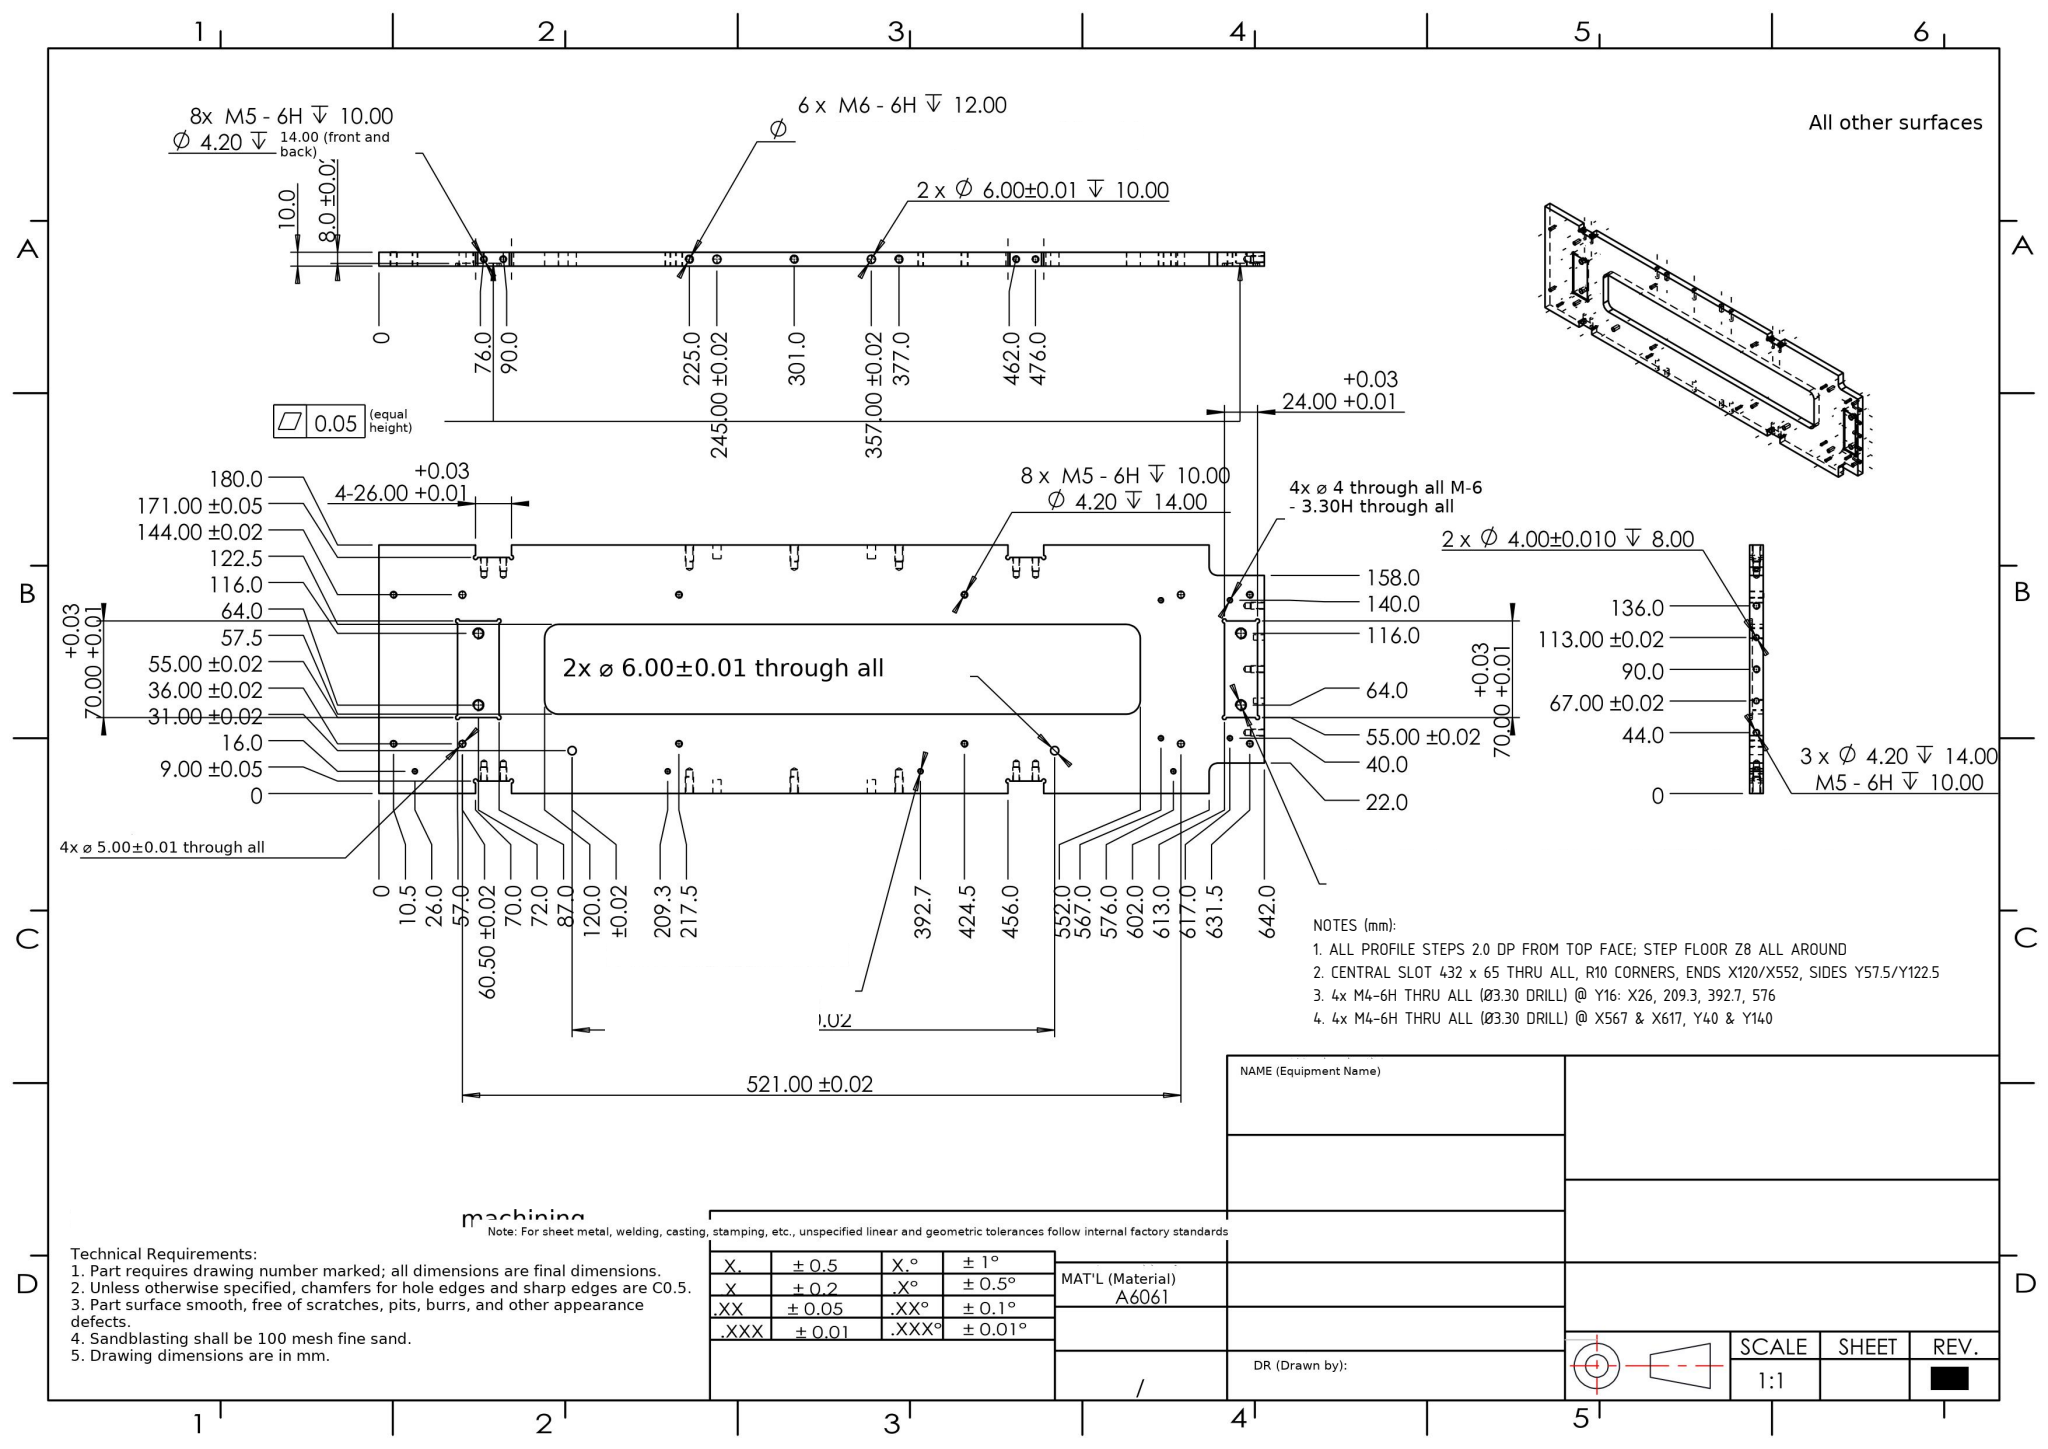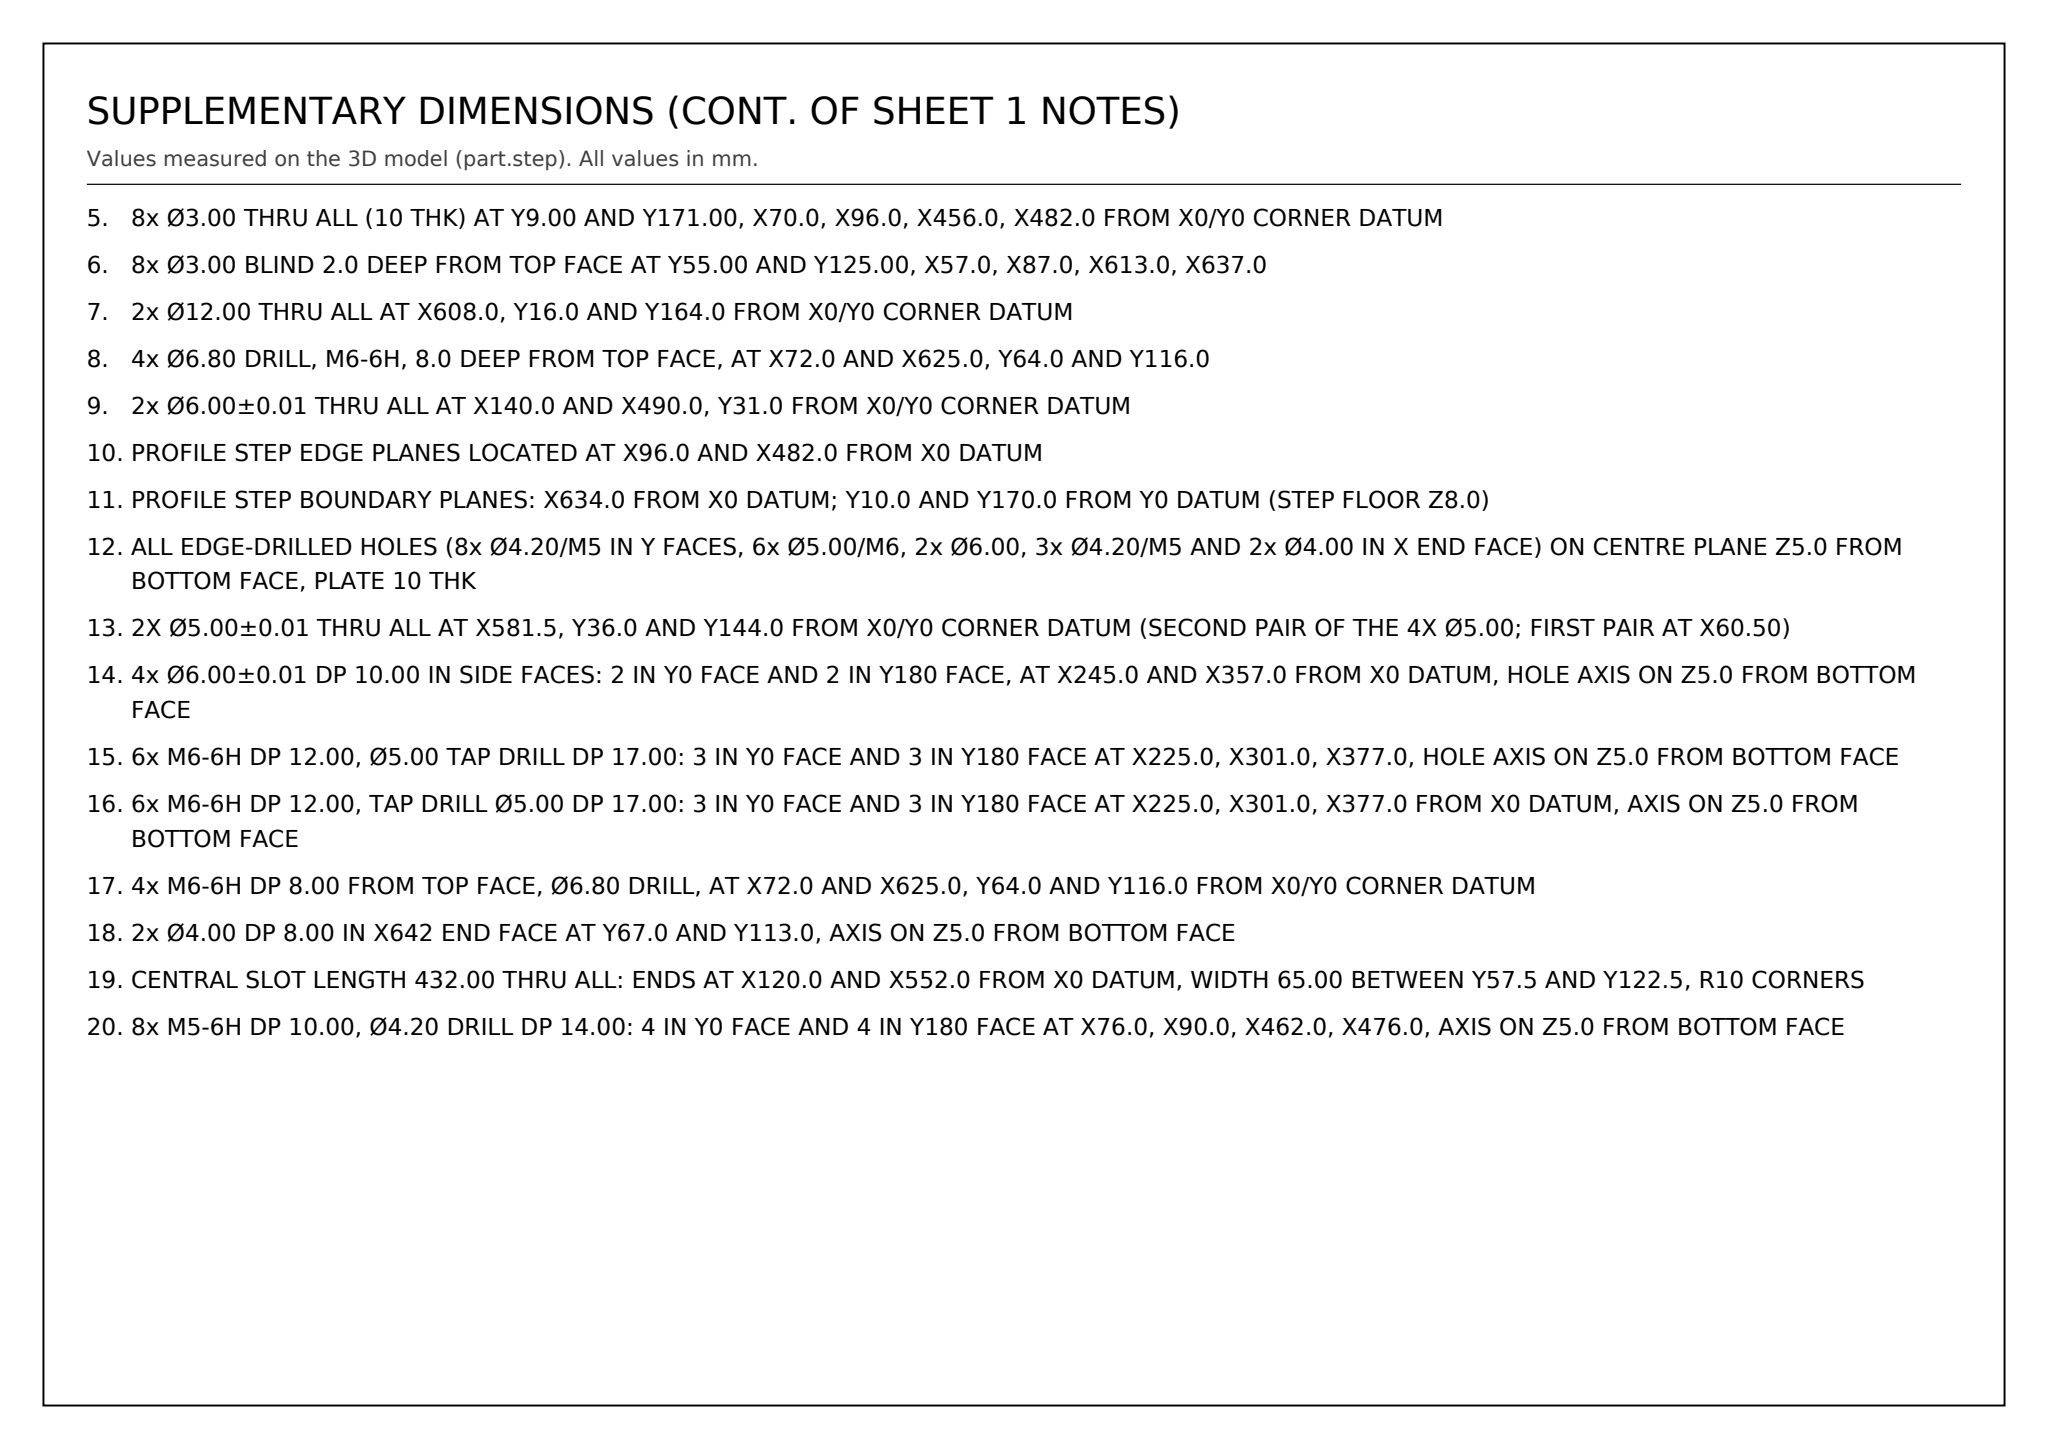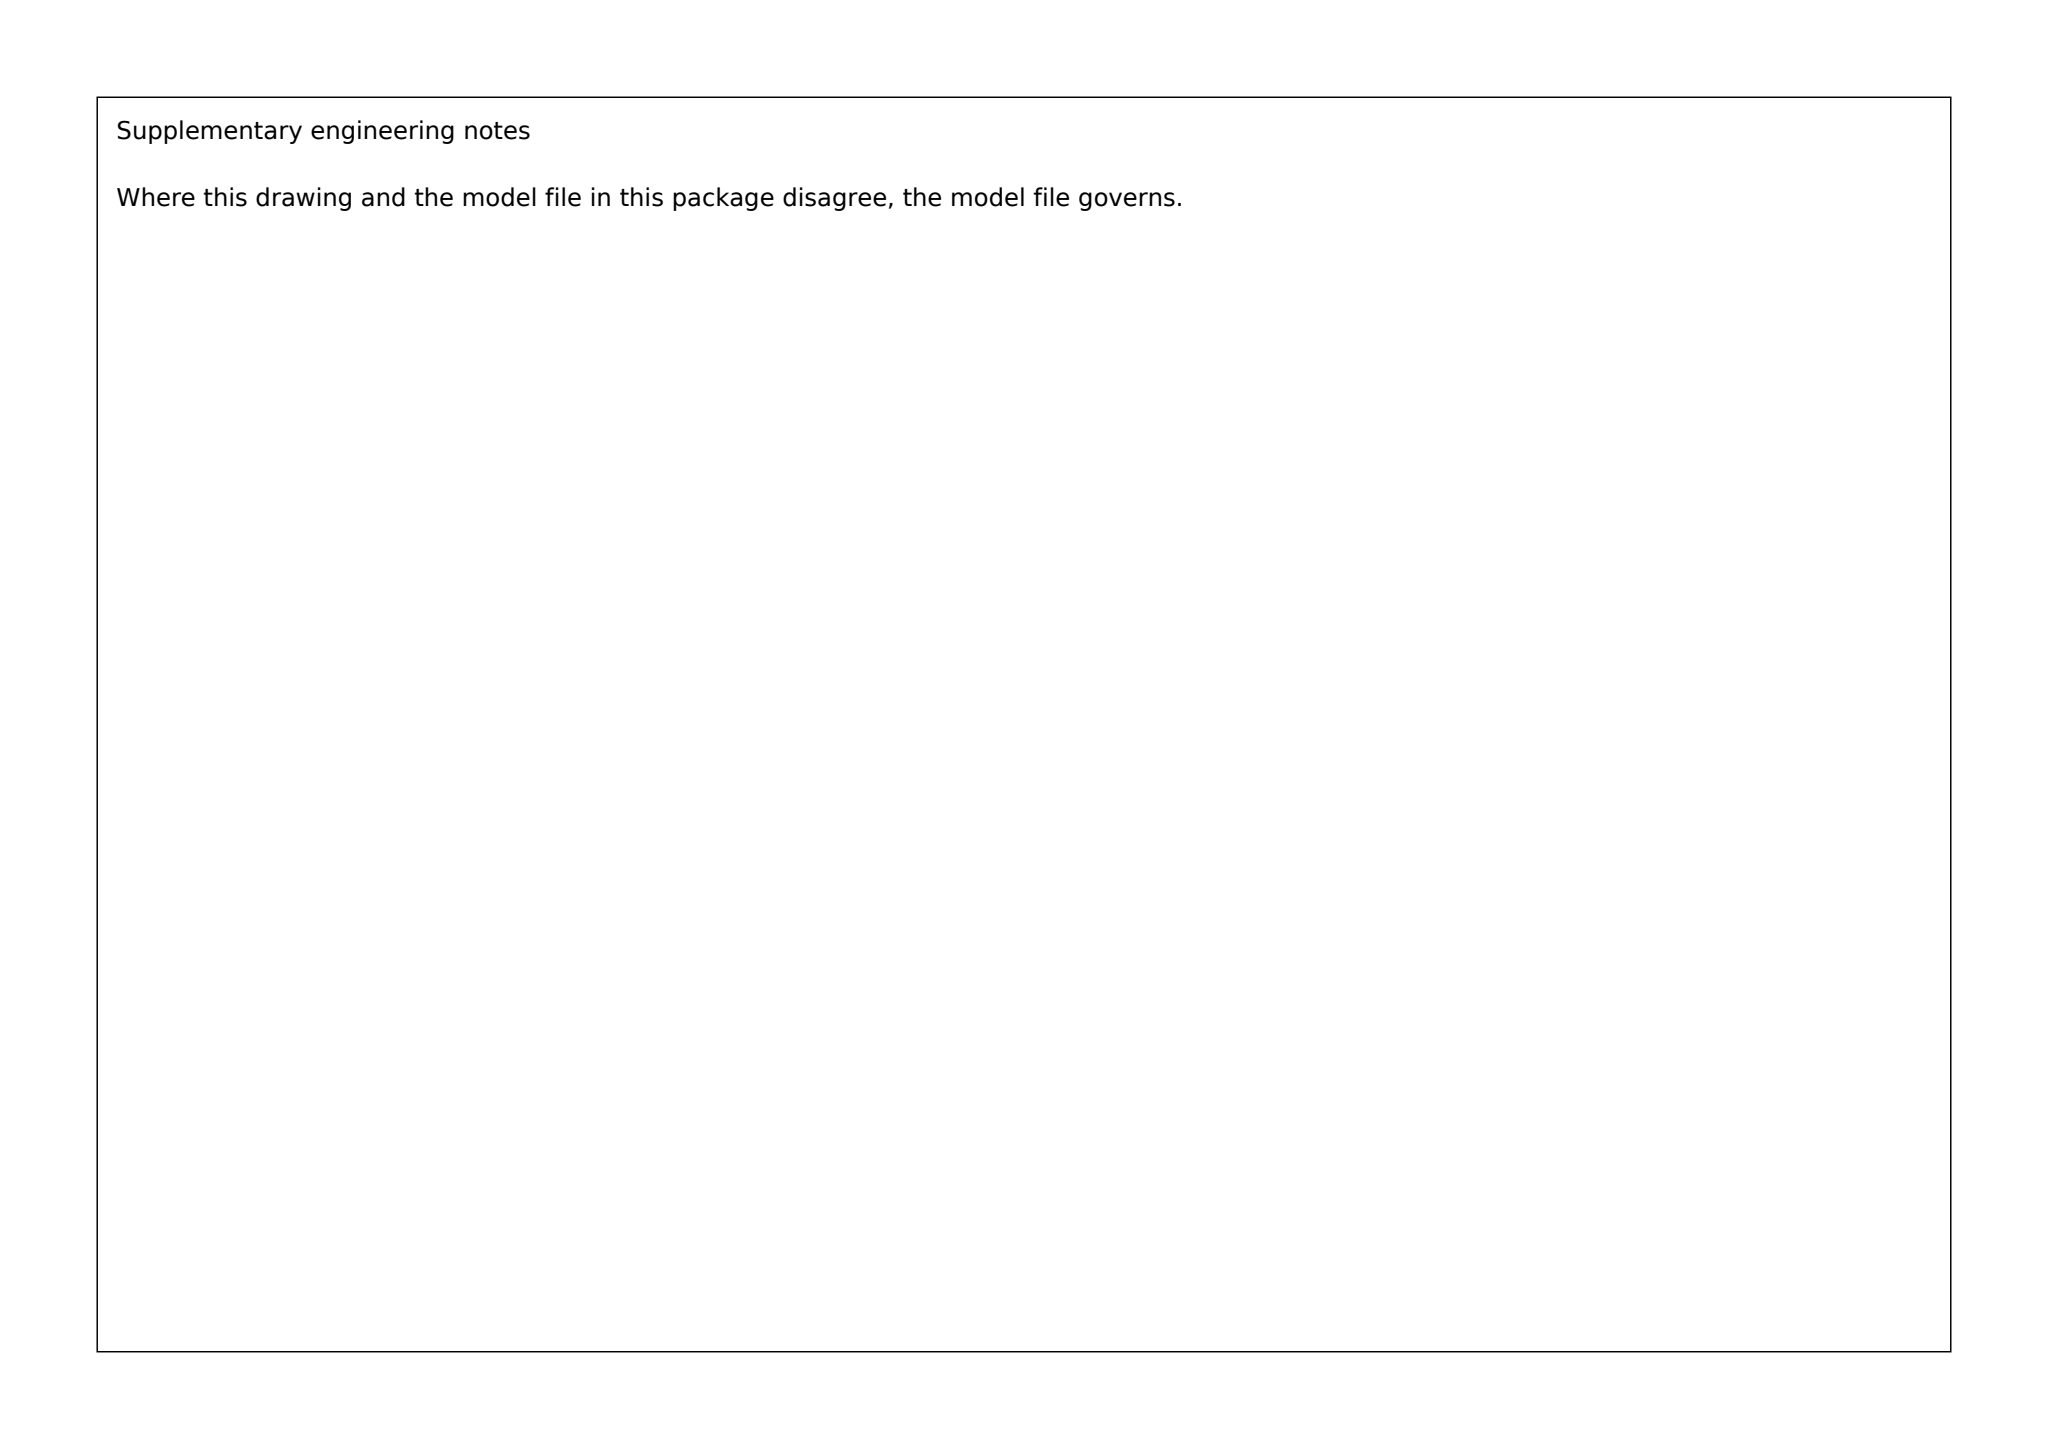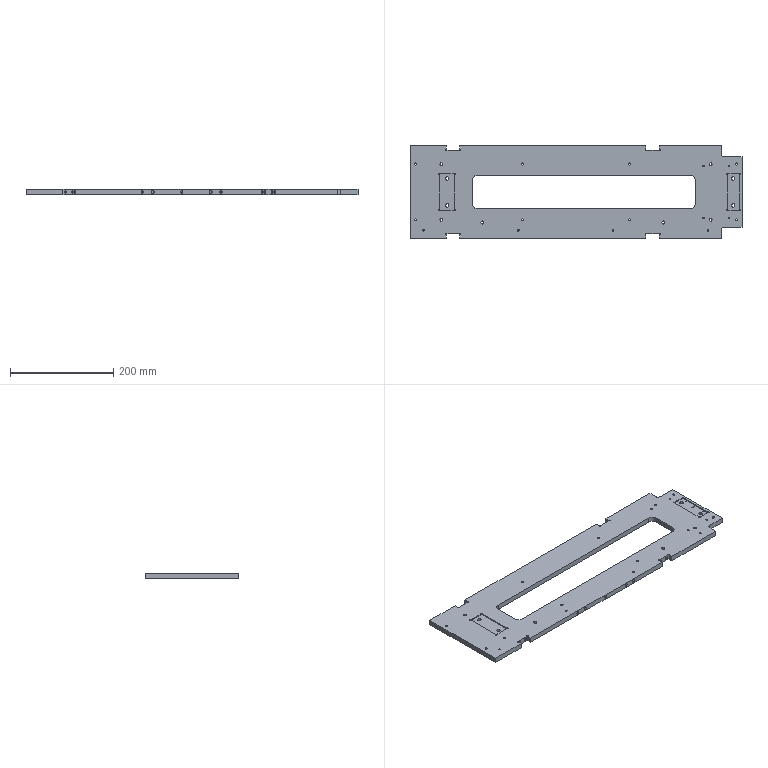Part | SolidWorks | mm | 1 solid | 208 faces | box 642 x 180 x 10 mm | volume 830887 mm3 | cylinder 128 | plane 46 | cone 34 | commonest cylinder face diameters 4.2 x38 3 x24 5 x20 3.3 x16 6 x12 6.8 x8 4 x4 20 x4
Drawing notes:
ALL PROFILE STEPS 2.0 DP FROM TOP FACE; STEP FLOOR Z8 ALL AROUND | from the solid: z planes 0, 8, 10 on 10 thk plate; floor at z=8
CENTRAL SLOT 432 x 65 THRU ALL, R10 CORNERS, ENDS X120/X552, SIDES Y57.5/Y122.5 | from the solid: x planes 120 & 552 (432), y planes 57.5 & 122.5 (65); R10 cyls Ø20 at (130,67.5),(130,112.5),(542,67.5),(542,112.5) len 10 = thru
4x M4-6H THRU ALL (Ø3.30 DRILL) @ Y16: X26, 209.3, 392.7, 576 | from the solid: Ø3.3 z-axis holes at (26,16),(209.33,16),(392.67,16),(576,16), len 10 = thru
4x M4-6H THRU ALL (Ø3.30 DRILL) @ X567 & X617, Y40 & Y140 | from the solid: Ø3.3 z-axis holes at (567,40),(567,140),(617,40),(617,140), len 10 = thru
8x Ø3.00 THRU ALL (10 THK) AT Y9.00 AND Y171.00, X70.0, X96.0, X456.0, X482.0 FROM X0/Y0 CORNER DATUM | from the solid: cylinders dia 3.0 axis z length 10.0 at (70,9),(70,171),(96,9),(96,171),(456,9),(456,171),(482,9),(482,171)
8x Ø3.00 BLIND 2.0 DEEP FROM TOP FACE AT Y55.00 AND Y125.00, X57.0, X87.0, X613.0, X637.0 | from the solid: cylinders dia 3.0 axis z length 2.0 at (57,55),(57,125),(87,55),(87,125),(613,55),(613,125),(637,55),(637,125)
2x Ø12.00 THRU ALL AT X608.0, Y16.0 AND Y164.0 FROM X0/Y0 CORNER DATUM | from the solid: cylinders dia 12.0 axis z length 10.0 at (608,16) and (608,164)
4x Ø6.80 DRILL, M6-6H, 8.0 DEEP FROM TOP FACE, AT X72.0 AND X625.0, Y64.0 AND Y116.0 | from the solid: cylinders dia 6.8 axis z length 8.0 at (72,64),(72,116),(625,64),(625,116)
2x Ø6.00±0.01 THRU ALL AT X140.0 AND X490.0, Y31.0 FROM X0/Y0 CORNER DATUM | from the solid: cylinders dia 6.0 axis z length 10.0 at (140,31) and (490,31)
PROFILE STEP EDGE PLANES LOCATED AT X96.0 AND X482.0 FROM X0 DATUM | from the solid: axis_planes normal x at offset 96.0 (2) and 482.0 (2)
PROFILE STEP BOUNDARY PLANES: X634.0 FROM X0 DATUM; Y10.0 AND Y170.0 FROM Y0 DATUM (STEP FLOOR Z8.0) | from the solid: axis_planes x 634.0 (2), y 10.0 (2), y 170.0 (2), z 8.0 (2)
ALL EDGE-DRILLED HOLES (8x Ø4.20/M5 IN Y FACES, 6x Ø5.00/M6, 2x Ø6.00, 3x Ø4.20/M5 AND 2x Ø4.00 IN X END FACE) ON CENTRE PLANE Z5.0 FROM BOTTOM FACE, PLATE 10 THK | from the solid: cylinders with axis x and axis y all have z position 5.0; bbox_xyz z = 10.0
2X Ø5.00±0.01 THRU ALL AT X581.5, Y36.0 AND Y144.0 FROM X0/Y0 CORNER DATUM (SECOND PAIR OF THE 4X Ø5.00; FIRST PAIR AT X60.50) | from the solid: cylinders [5.0, z, (581.5, 36.0), len 10.0] and [5.0, z, (581.5, 144.0), len 10.0] in 10 THK plate
4x Ø6.00±0.01 DP 10.00 IN SIDE FACES: 2 IN Y0 FACE AND 2 IN Y180 FACE, AT X245.0 AND X357.0 FROM X0 DATUM, HOLE AXIS ON Z5.0 FROM BOTTOM FACE | from the solid: cylinders dia 6.0 axis y at [245.0,*,5.0] from y0 to y10 and from y170 to y180; same at [357.0,*,5.0]
6x M6-6H DP 12.00, Ø5.00 TAP DRILL DP 17.00: 3 IN Y0 FACE AND 3 IN Y180 FACE AT X225.0, X301.0, X377.0, HOLE AXIS ON Z5.0 FROM BOTTOM FACE | from the solid: cylinders dia 5.0 axis y at [225.0/301.0/377.0,*,5.0] from y0 to y17 and from y163 to y180
6x M6-6H DP 12.00, TAP DRILL Ø5.00 DP 17.00: 3 IN Y0 FACE AND 3 IN Y180 FACE AT X225.0, X301.0, X377.0 FROM X0 DATUM, AXIS ON Z5.0 FROM BOTTOM FACE | from the solid: cylinders: hole/bore Ø5.0 axis y at X225.0/X301.0/X377.0, z=5.0, ranges 0->17 and 163->180
4x M6-6H DP 8.00 FROM TOP FACE, Ø6.80 DRILL, AT X72.0 AND X625.0, Y64.0 AND Y116.0 FROM X0/Y0 CORNER DATUM | from the solid: cylinders: hole/bore Ø6.8 axis z at (72,116),(72,64),(625,116),(625,64) from z0 to z8
2x Ø4.00 DP 8.00 IN X642 END FACE AT Y67.0 AND Y113.0, AXIS ON Z5.0 FROM BOTTOM FACE | from the solid: cylinders: hole/bore Ø4.0 axis x at y=67.0 and y=113.0, z=5.0, from X634.0 to X642.0
CENTRAL SLOT LENGTH 432.00 THRU ALL: ENDS AT X120.0 AND X552.0 FROM X0 DATUM, WIDTH 65.00 BETWEEN Y57.5 AND Y122.5, R10 CORNERS | from the solid: axis_planes x=120.0 and x=552.0 (y 67.5-112.5, z 0-10) with R10 concave arcs at (130,112.5),(130,67.5),(542,112.5),(542,67.5) z0->10
8x M5-6H DP 10.00, Ø4.20 DRILL DP 14.00: 4 IN Y0 FACE AND 4 IN Y180 FACE AT X76.0, X90.0, X462.0, X476.0, AXIS ON Z5.0 FROM BOTTOM FACE | from the solid: cylinders: hole/bore Ø4.2 axis y at X76.0/X90.0/X462.0/X476.0, z=5.0, ranges 9->23 and 157->171 (14.0 deep)